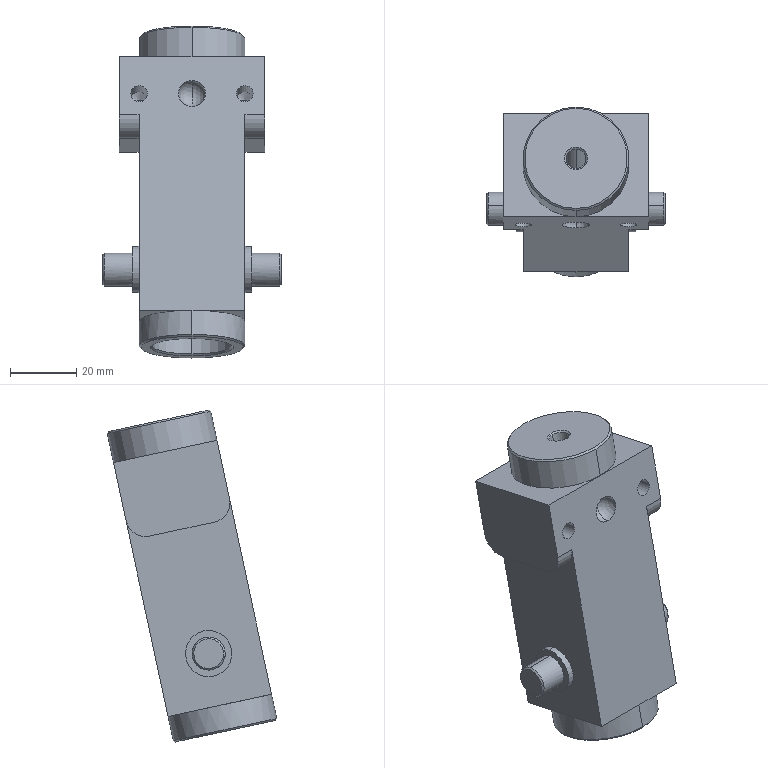Component | SolidWorks | Ornament-1 | 1 solid | 64 faces | box 54 x 51.24 x 100.37 mm | volume 75883 mm3 | cylinder 24 | plane 20 | cone 18 | sphere 2 | commonest cylinder face diameters 5 x4 10 x4 14 x4 32 x4 12 x4 6 x2 24 x2
build123d program:
from build123d import *

# Parameters (mm, degrees)
SKETCH1_2_W                   = 32
SKETCH1_2_H                   = 78.5
BOSS_EXTRUDE1_DEPTH           = 32
SKETCH2_R                     = 16
BOSS_EXTRUDE2_DEPTH           = 9.5
BOSS_EXTRUDE3_START           = 8
SKETCH3_R                     = 16
BOSS_EXTRUDE3_DEPTH           = 8
SKETCH4_W                     = 32
SKETCH4_H                     = 24
BOSS_EXTRUDE4_DEPTH           = 6
FILLET1_R                     = 6
FILLET1_OF_MIRROR1_R          = 6
SKETCH5_R                     = 7
BOSS_EXTRUDE5_DEPTH           = 2
SKETCH6_R                     = 5
BOSS_EXTRUDE6_DEPTH           = 9
SIZE_MM_DOWEL_PIN_HOLE1_D     = 24
SIZE_MM_DOWEL_PIN_HOLE1_DEPTH = 60
SIZE_MM_DOWEL_PIN_HOLE1_TIP   = 7.21
SIZE_MM_DOWEL_PIN_HOLE2_D     = 6
M6_TAPPED_HOLE1_D             = 5
M6_TAPPED_HOLE1_DEPTH         = 9
M6_TAPPED_HOLE1_TIP           = 1.502
CHAMFER1_SIZE                 = 0.5


with BuildPart() as part:
    # Sketch1_2 → Boss-Extrude1 (new body)
    with BuildSketch(Plane.XY):
        Rectangle(SKETCH1_2_W, SKETCH1_2_H)
    extrude(amount=BOSS_EXTRUDE1_DEPTH)

    # Sketch2 → Boss-Extrude2 (add)
    with BuildSketch(Plane(origin=(0, 39.25, 0), x_dir=(1, 0, 0), z_dir=(0, 1, 0))):
        with Locations(Location((0, -16, 0), (0, 0, 270))):
            Circle(SKETCH2_R)
    extrude(amount=BOSS_EXTRUDE2_DEPTH)

    # Sketch3 → Boss-Extrude3 (add)
    with BuildSketch(Plane.XZ.offset(39.25).offset(BOSS_EXTRUDE3_START)):
        with Locations(Location((0, 16, 0), (0, 0, 90))):
            Circle(SKETCH3_R)
    extrude(amount=-BOSS_EXTRUDE3_DEPTH)

    # Sketch4 → Boss-Extrude4 (add)
    with BuildSketch(Plane.ZY.offset(16)):
        with Locations((16, 27.25)):
            Rectangle(SKETCH4_W, SKETCH4_H)
    boss_extrude4 = extrude(amount=BOSS_EXTRUDE4_DEPTH)

    # Fillet1
    fillet1_edges = [part.edges().sort_by_distance(p)[0] for p in [
        (-19, 15.25, 0),
        (-19, 15.25, 32),
    ]]
    fillet(fillet1_edges, radius=FILLET1_R)

    # Mirror1: Boss-Extrude4 across plane
    add(boss_extrude4.mirror(Plane.ZY))

    # Fillet1 of Mirror1
    fillet1_of_mirror1_edges = [part.edges().sort_by_distance(p)[0] for p in [
        (19, 15.25, 0),
        (19, 15.25, 32),
    ]]
    fillet(fillet1_of_mirror1_edges, radius=FILLET1_OF_MIRROR1_R)

    # Sketch5 → Boss-Extrude5 (add)
    with BuildSketch(Plane.ZY.offset(16)):
        with Locations(Location((16, -23.25, 0), (0, 0, 90))):
            Circle(SKETCH5_R)
    boss_extrude5 = extrude(amount=BOSS_EXTRUDE5_DEPTH)

    # Sketch6 → Boss-Extrude6 (add)
    with BuildSketch(Plane.ZY.offset(18)):
        with Locations(Location((16, -23.25, 0), (0, 0, 270))):
            Circle(SKETCH6_R)
    boss_extrude6 = extrude(amount=BOSS_EXTRUDE6_DEPTH)

    # Mirror2: Boss-Extrude5, Boss-Extrude6 across plane
    add(boss_extrude5.mirror(Plane.ZY))
    add(boss_extrude6.mirror(Plane.ZY))

    # Size mm Dowel Pin Hole1
    with Locations(Plane(origin=(0, -47.25, 0), x_dir=(-1, 0, 0), z_dir=(0, -1, 0))):
        with Locations((0, -16)):
            Hole(SIZE_MM_DOWEL_PIN_HOLE1_D / 2, depth=SIZE_MM_DOWEL_PIN_HOLE1_DEPTH)
            with Locations((0, 0, -(SIZE_MM_DOWEL_PIN_HOLE1_DEPTH + SIZE_MM_DOWEL_PIN_HOLE1_TIP / 2))):  # 118° drill point
                Cone(0, SIZE_MM_DOWEL_PIN_HOLE1_D / 2, SIZE_MM_DOWEL_PIN_HOLE1_TIP, mode=Mode.SUBTRACT)

    # Size mm Dowel Pin Hole2 (through all)
    with Locations(Plane(origin=(0, 48.75, 0), x_dir=(1, 0, 0), z_dir=(0, 1, 0))):
        with Locations((0, -16)):
            Hole(SIZE_MM_DOWEL_PIN_HOLE2_D / 2)

    # Sketch13 → Cut-Revolve1 (revolve, cut)
    with BuildSketch(Plane.ZY):
        with BuildLine():
            Line((0, 31.8), (0, 23.7))
            ThreePointArc((0, 23.7), (4.05, 27.75), (0, 31.8))
        make_face()
    revolve(axis=Axis((0, 31.8, 0), (0, -1, 0)), mode=Mode.SUBTRACT)

    # M6 Tapped Hole1
    with Locations(Plane(origin=(0, 0, 0), x_dir=(-1, 0, 0), z_dir=(0, 0, -1))):
        with Locations((-16, 27.75), (16, 27.75)):
            Hole(M6_TAPPED_HOLE1_D / 2, depth=M6_TAPPED_HOLE1_DEPTH)
            with Locations((0, 0, -(M6_TAPPED_HOLE1_DEPTH + M6_TAPPED_HOLE1_TIP / 2))):  # 118° drill point
                Cone(0, M6_TAPPED_HOLE1_D / 2, M6_TAPPED_HOLE1_TIP, mode=Mode.SUBTRACT)

    # Chamfer1
    chamfer1_edges = [part.edges().sort_by_distance(p)[0] for p in [
        (-27, -18.25, 16),
        (27, -18.25, 16),
        (-12, -47.25, 16),
        (3, 48.75, 16),
        (0, 48.75, 0),
        (0, -47.25, 0),
    ]]
    chamfer(chamfer1_edges, length=CHAMFER1_SIZE)


solid = part.part

# Placed as in the assembly
solid = solid.moved(Location((111.296, 66.242, 464.764), (-102.127, 0, -180)))